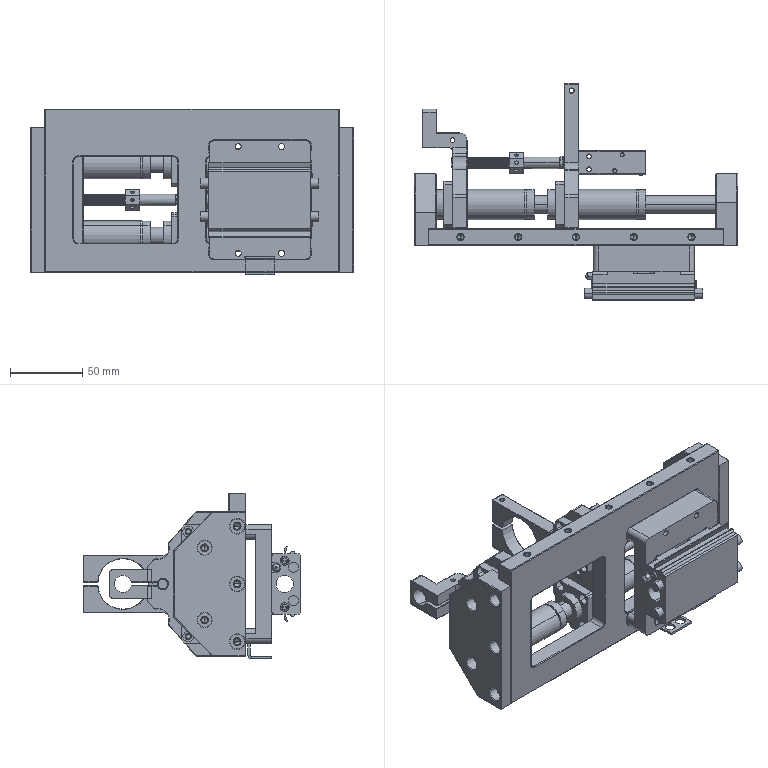Assembly | SolidWorks | mm | 23 component files | 23 solids | 1814 faces | box 224 x 150.5 x 115 mm | volume 625132 mm3 | cylinder 845 | plane 504 | cone 226 | torus 172 | spline 66 | sphere 1 | commonest cylinder face diameters 8 x107 0.4 x84 6 x62 4.2 x50 1 x50 3.3 x42 10 x38 4.5 x38
Bill of materials:
D12-200 | 2 |  | Long slender straight cylindrical tube with a small central bore and a thick wall.
KK60-A0 | 1 |  | Rectangular block body with two short cylindrical pins sticking out of each end face, a large round opening through the end face, and long grooves/ribs along the top and bottom long faces.
KKConnectingPlate-3 | 1 |  | Rectangular plate with rounded corners and a C-shaped section: a thick face with flanges at two opposite edges, drilled with eight through holes and with a rectangular notch in one edge.
LHFRW_MX12 | 4 |  | Hollow cylindrical tube with a through bore and a square flange with chamfered corners and four corner through-holes. The flange sits close to one end, so a short section of the cylinder sticks out behind it. Narrow circumferential grooves or steps sit next to the flange and near the far end of the long body.
NozzleConnectingPost | 1 |  | Hollow cylindrical threaded sleeve or stud with three sections: a long externally threaded section, a short section of smaller diameter that also looks threaded with a flat, and a plain smooth section with an open bore at the end.
NozzleFixingPlate | 1 |  | Flat bracket plate with two large round holes, each surrounded by four small holes. The outline has angled edges and concave scallops, and an arm turns off the plate as an offset tab ending in a split clamp ring.
Nut | 1 |  | Octagonal prism block with a large central through bore along its axis and small radial cross holes in the side faces.
Z-AxisElectricScrewdriverBasePlate | 1 |  | Flat rectangular frame plate with two rectangular windows with rounded corners. One window has a shallow recessed slot above it and one below it, each slot holding three holes. The plate edges carry rows of holes.
Z-AxisElectricScrewdriverFixingPlate | 1 |  | Flat bracket plate with angled corners and an extended arm that ends in a large split clamp bore. The main body has two large holes, each with four small holes around it, plus two medium holes.
Z-AxisElectricScrewdriverFixingPlateBottomPlate | 1 |  | Thick plate with a stepped (rabbeted) section along one long edge and two chamfered corners on the opposite side. It has three plain holes in the narrow stepped strip and two counterbored holes in the main area.
Z-AxisElectricScrewdriverFixingPlateTopPlate | 1 |  | Thick plate with chamfered corners on one side and a stepped edge profile, with six counterbored through holes in two staggered columns.
Z-AxisSpringGuidePost | 1 |  | Long straight cylindrical tube with a relatively thin wall and a large concentric bore.
ZSensorPiece | 1 |  | Bent sheet-like U/C-shaped bracket: two parallel flat legs joined by a web with a generous bend radius. One leg has two obround slots and the other has two round holes.
Mates:
1. concentric | KK60-A0-1 face at (-38.981, 23.016, 97) dir (0, 1, 0) r 2.1 | KKConnectingPlate-3-1 face at (-38.981, 33.016, 97) dir (0, 1, 0) r 5
2. concentric | KK60-A0-1 face at (-38.981, 23.016, 67) dir (0, 1, 0) r 2.1 | KKConnectingPlate-3-1 face at (-38.981, 33.016, 67) dir (0, 1, 0) r 2.75
3. coincident | KK60-A0-1 face at (-59.481, 23.016, 61) dir (0, 1, 0) | KKConnectingPlate-3-1 face at (55.019, 23.016, 82) dir (0, -1, 0)
4. concentric | KKConnectingPlate-3-1 face at (-8.981, 42.016, 45) dir (0, 1, 0) r 2.1 | Z-AxisElectricScrewdriverBasePlate-1 face at (-8.981, 52.016, 45) dir (0, 1, 0) r 5.5
5. concentric | KKConnectingPlate-3-1 face at (-38.981, 42.016, 45) dir (0, 1, 0) r 2.1 | Z-AxisElectricScrewdriverBasePlate-1 face at (-38.981, 52.016, 45) dir (0, 1, 0) r 5.5
6. coincident | KKConnectingPlate-3-1 face at (-58.981, 42.016, 113) dir (0, 1, 0) | Z-AxisElectricScrewdriverBasePlate-1 face at (-172.981, 42.016, 132) dir (0, -1, 0)
7. coincident | Z-AxisElectricScrewdriverBasePlate-1 face at (31.019, 40.016, 132) dir (1, 0, 0) | Z-AxisElectricScrewdriverFixingPlateTopPlate-1 face at (31.019, 40.016, 32) dir (-1, 0, 0)
8. concentric | Z-AxisElectricScrewdriverBasePlate-1 edge at (-172.981, 46.016, 42) dir (-1, 0, 0) r 2.525 | Z-AxisElectricScrewdriverFixingPlateBottomPlate-1 face at (-182.981, 46.016, 42) dir (-1, 0, 0) r 2.75
9. coincident | Z-AxisElectricScrewdriverBasePlate-1 face at (-172.981, 40.016, 32) dir (-1, 0, 0) | Z-AxisElectricScrewdriverFixingPlateBottomPlate-1 face at (-172.981, 52.016, 32) dir (1, 0, 0)
10. coincident | Z-AxisElectricScrewdriverFixingPlateTopPlate-1 face at (29.019, 68.516, 54.25) dir (-1, 0, 0) | D12-200-1 face at (29.019, 68.516, 57) dir (1, 0, 0)
11. coincident | Z-AxisElectricScrewdriverFixingPlateTopPlate-1 face at (29.019, 68.516, 104.25) dir (-1, 0, 0) | D12-200-2 face at (29.019, 68.516, 107) dir (1, 0, 0)
12. concentric | Z-AxisElectricScrewdriverFixingPlateBottomPlate-1 face at (-182.981, 68.516, 57) dir (1, 0, 0) r 6.05 | D12-200-1 face at (29.019, 68.516, 57) dir (-1, 0, 0) r 6
13. concentric | Z-AxisElectricScrewdriverFixingPlateBottomPlate-1 face at (-182.981, 68.516, 107) dir (1, 0, 0) r 6.05 | D12-200-2 face at (29.019, 68.516, 107) dir (-1, 0, 0) r 6
14. coincident | Z-AxisElectricScrewdriverFixingPlateTopPlate-1 face at (29.019, 68.516, 79.25) dir (-1, 0, 0) | Z-AxisSpringGuidePost-1 face at (29.019, 68.516, 82) dir (1, 0, 0)
15. concentric | D12-200-1 face at (29.019, 68.516, 57) dir (-1, 0, 0) r 6 | LHFRW_MX12-1 face at (-27.981, 68.516, 57) dir (-1, 0, 0) r 10.5
16. concentric | D12-200-2 face at (29.019, 68.516, 107) dir (-1, 0, 0) r 6 | LHFRW_MX12-2 face at (-27.981, 68.516, 107) dir (-1, 0, 0) r 10.5
17. coincident | LHFRW_MX12-1 face at (-22.481, 84.516, 41) dir (0, 1, 0) | LHFRW_MX12-2 face at (-22.481, 84.516, 91) dir (0, 1, 0)
18. coincident | Z-AxisElectricScrewdriverFixingPlate-1 face at (-78.981, 52.516, 132) dir (-1, 0, 0) | LHFRW_MX12-1 face at (-78.981, 75.728, 64.212) dir (1, 0, 0)
19. concentric | Z-AxisElectricScrewdriverFixingPlate-1 face at (-78.981, 68.516, 107) dir (-1, 0, 0) r 10.5 | LHFRW_MX12-2 face at (-27.981, 68.516, 107) dir (-1, 0, 0) r 10.5
20. concentric | Z-AxisElectricScrewdriverFixingPlate-1 face at (-78.981, 68.516, 57) dir (-1, 0, 0) r 10.5 | LHFRW_MX12-1 face at (-27.981, 68.516, 57) dir (-1, 0, 0) r 10.5
21. coincident | Z-AxisElectricScrewdriverFixingPlate-1 face at (-78.981, 52.516, 132) dir (-1, 0, 0) | LHFRW_MX12-2 face at (-78.981, 75.728, 114.212) dir (1, 0, 0)
22. concentric | D12-200-1 face at (29.019, 68.516, 57) dir (-1, 0, 0) r 6 | NozzleFixingPlate-1 face at (-146.481, 68.516, 57) dir (1, 0, 0) r 10.5
23. concentric | D12-200-2 face at (29.019, 68.516, 107) dir (-1, 0, 0) r 6 | NozzleFixingPlate-1 face at (-146.481, 68.516, 107) dir (1, 0, 0) r 10.5
24. concentric | D12-200-1 face at (29.019, 68.516, 57) dir (-1, 0, 0) r 6 | LHFRW_MX12-3 face at (-105.481, 68.516, 57) dir (-1, 0, 0) r 10.5
25. concentric | D12-200-2 face at (29.019, 68.516, 107) dir (-1, 0, 0) r 6 | LHFRW_MX12-4 face at (-105.481, 68.516, 107) dir (-1, 0, 0) r 10.5
26. coincident | LHFRW_MX12-3 face at (-162.481, 83.365, 71.849) dir (-1, 0, 0) | LHFRW_MX12-4 face at (-162.481, 83.365, 121.849) dir (-1, 0, 0)
27. coincident | LHFRW_MX12-3 face at (-99.981, 84.516, 41) dir (0, 1, 0) | LHFRW_MX12-4 face at (-99.981, 84.516, 91) dir (0, 1, 0)
28. coincident | NozzleFixingPlate-1 face at (-156.481, 97.516, 82) dir (-1, 0, 0) | LHFRW_MX12-3 face at (-156.481, 75.728, 64.212) dir (1, 0, 0)
29. coincident | Z-AxisSpringGuidePost-1 face at (-78.981, 68.516, 82) dir (-1, 0, 0) | Z-AxisElectricScrewdriverFixingPlate-1 face at (-78.981, 52.516, 132) dir (-1, 0, 0)
30. coincident | Z-AxisElectricScrewdriverFixingPlateBottomPlate-1 face at (-167.981, 90.016, 32) dir (1, 0, 0) | LHFRW_MX12-3 face at (-167.981, 75.87, 64.354) dir (-1, 0, 0)
31. coincident | KKConnectingPlate-3-1 face at (55.019, 23.016, 43) dir (0, 0, -1) | ZSensorPiece-1 face at (-23.981, 29.516, 43) dir (0, 0, 1)
32. concentric | Z-AxisElectricScrewdriverFixingPlate-1 edge at (-69.181, 97.516, 73) dir (1, 0, 0) r 1.7 | MD-10x10-S-G1-2 (0)-1/MD 10x10-S10 - Body-1 edge at (-68.981, 97.516, 73) dir (-1, 0, 0) r 1.5
33. concentric | Z-AxisElectricScrewdriverFixingPlate-1 face at (-68.981, 97.516, 82) dir (-1, 0, 0) r 5 | MD-10x10-S-G1-2 (0)-1/MD 10x10-S10 - Rod-1 face at (-31.981, 97.516, 82) dir (-1, 0, 0) r 2
34. coincident | Z-AxisElectricScrewdriverFixingPlate-1 face at (-68.981, 52.516, 132) dir (1, 0, 0) | MD-10x10-S-G1-2 (0)-1/MD 10x10-S10 - Body-1 face at (-68.981, 105.466, 91.1) dir (-1, 0, 0)
35. concentric | MD-10x10-S-G1-2 (0)-1/MD 10x10-S10 - Rod-1 face at (-31.981, 97.516, 82) dir (-1, 0, 0) r 2 | NozzleConnectingPost-1 face at (-82.181, 97.516, 82) dir (-1, 0, 0) r 4
36. coincident | MD-10x10-S-G1-2 (0)-1/MD 10x10 - Nut Rod-1 face at (-82.181, 94.016, 82) dir (-1, 0, 0) | NozzleConnectingPost-1 face at (-82.181, 97.516, 82) dir (1, 0, 0)
37. coincident | NozzleConnectingPost-1 face at (-107.181, 107.516, 79) dir (-1, 0, 0) | Nut-1 face at (-107.181, 97.516, 82) dir (1, 0, 0)
38. concentric | Z-AxisElectricScrewdriverBasePlate-1 face at (31.019, 46.016, 42) dir (-1, 0, 0) r 785.398 | Z-AxisElectricScrewdriverFixingPlateTopPlate-1 face at (41.019, 46.016, 42) dir (1, 0, 0) r 2.75
39. concentric | Z-AxisElectricScrewdriverBasePlate-1 face at (31.019, 46.016, 82) dir (1, 0, 0) r 2.1 | Z-AxisElectricScrewdriverFixingPlateTopPlate-1 face at (41.019, 46.016, 82) dir (1, 0, 0) r 2.75
40. concentric | Z-AxisSpringGuidePost-1 face at (29.019, 68.516, 82) dir (-1, 0, 0) r 4 | Z-AxisElectricScrewdriverFixingPlate-1 face at (-68.981, 68.516, 82) dir (1, 0, 0) r 4.05
41. concentric | KKConnectingPlate-3-1 face at (-18.981, 32.016, 43) dir (0, 0, -1) r 1.65 | ZSensorPiece-1 face at (-18.981, 32.016, 51.5) dir (0, 0, -1) r 2.25
42. concentric | KKConnectingPlate-3-1 face at (-28.981, 32.016, 43) dir (0, 0, -1) r 1.65 | ZSensorPiece-1 face at (-28.981, 32.016, 51.5) dir (0, 0, -1) r 2.25
43. coincident | Z-AxisElectricScrewdriverBasePlate-1 face at (-172.981, 52.016, 132) dir (0, 1, 0) | Z-AxisElectricScrewdriverFixingPlateBottomPlate-1 face at (-167.981, 52.016, 32) dir (0, -1, 0)
44. concentric | NozzleConnectingPost-1 face at (-82.181, 97.516, 82) dir (-1, 0, 0) r 4 | Nut-1 face at (-117.181, 97.516, 82) dir (1, 0, 0) r 4
45. coincident | MD 10x10-S10 - Body-1 axis at (80.9, 0, 0) dir (-1, 0, 0) | MD 10x10-S10 - Rod-1 axis at (80.9, 0, 0) dir (-1, 0, 0)
46. angle | MD 10x10-S10 - Rod-1 plane at (0, 0, 0) dir (0, 1, 0) | MD 10x10-S10 - Body-1 plane at (0, 0, 0) dir (0, 0, -1)
47. coincident | MD 10x10-S10 - Rod-1 axis at (-80.9, 0, 0) dir (1, 0, 0) | MD 10x10 - Nut Rod-1 axis at (-91.9, 0, 0) dir (1, 0, 0)
48. angle | MD 10x10 - Nut Rod-1 plane at (-11, 0, 0) dir (0, 1, 0) | MD 10x10-S10 - Rod-1 plane at (0, 0, 0) dir (0, 1, 0)
49. coincident | MD 10x10-S10 - Rod-1 axis at (-80.9, 0, 0) dir (1, 0, 0) | MD 10x10 - Nut Rod-2 axis at (69.9, 0, 0) dir (-1, 0, 0)
50. angle | MD 10x10 - Nut Rod-2 plane at (-11, 0, 0) dir (0, 1, 0) | MD 10x10-S10 - Rod-1 plane at (0, 0, 0) dir (0, 1, 0)